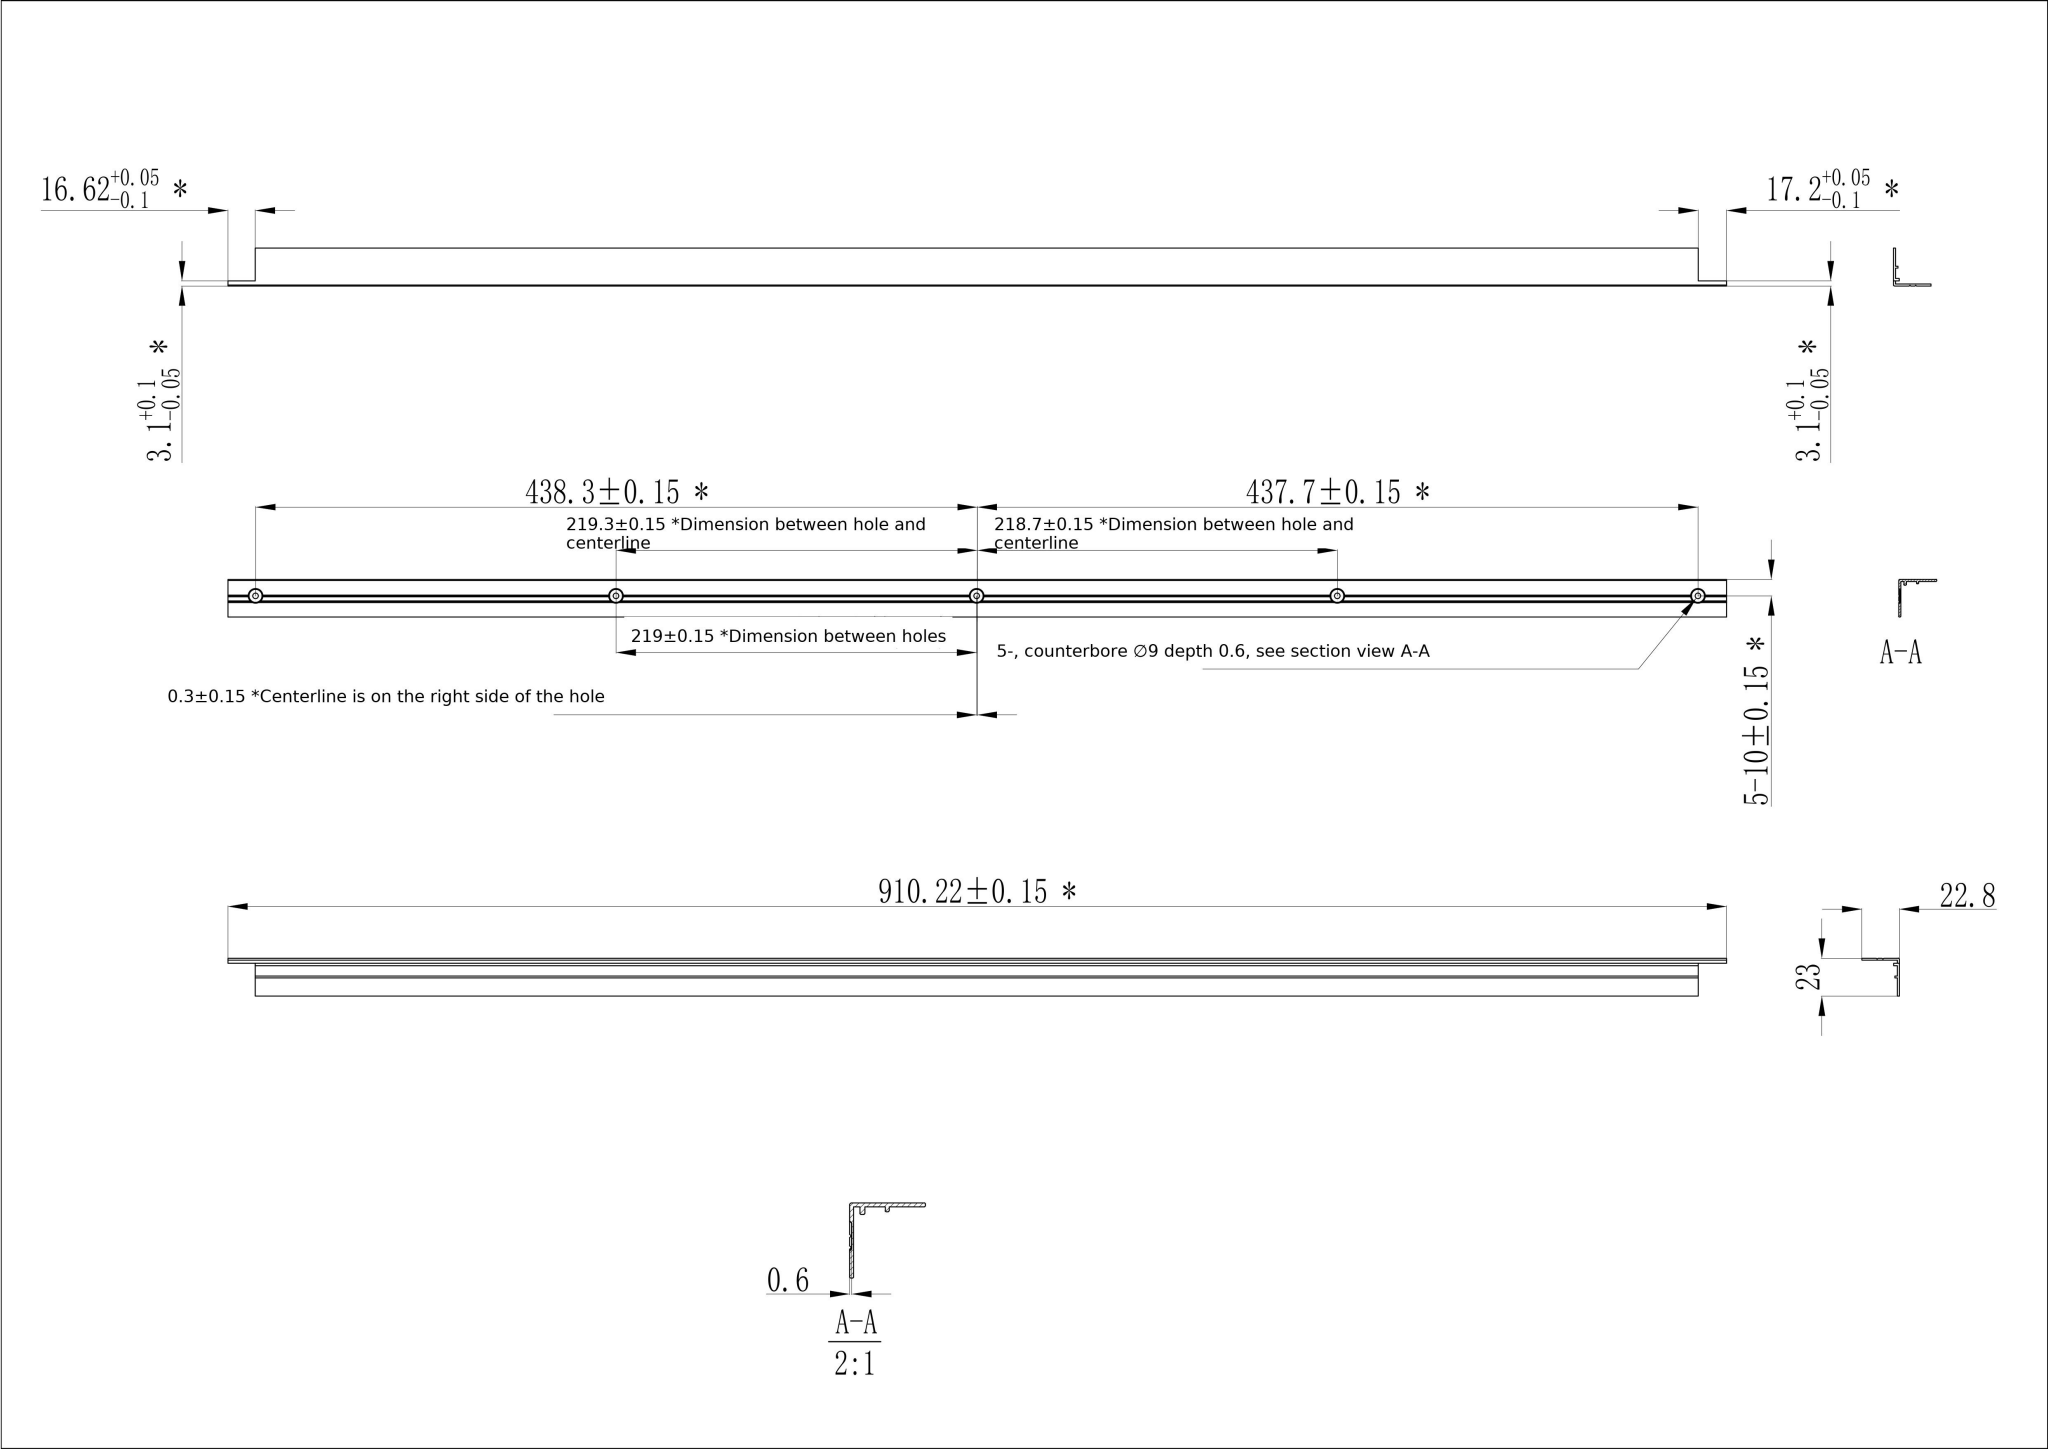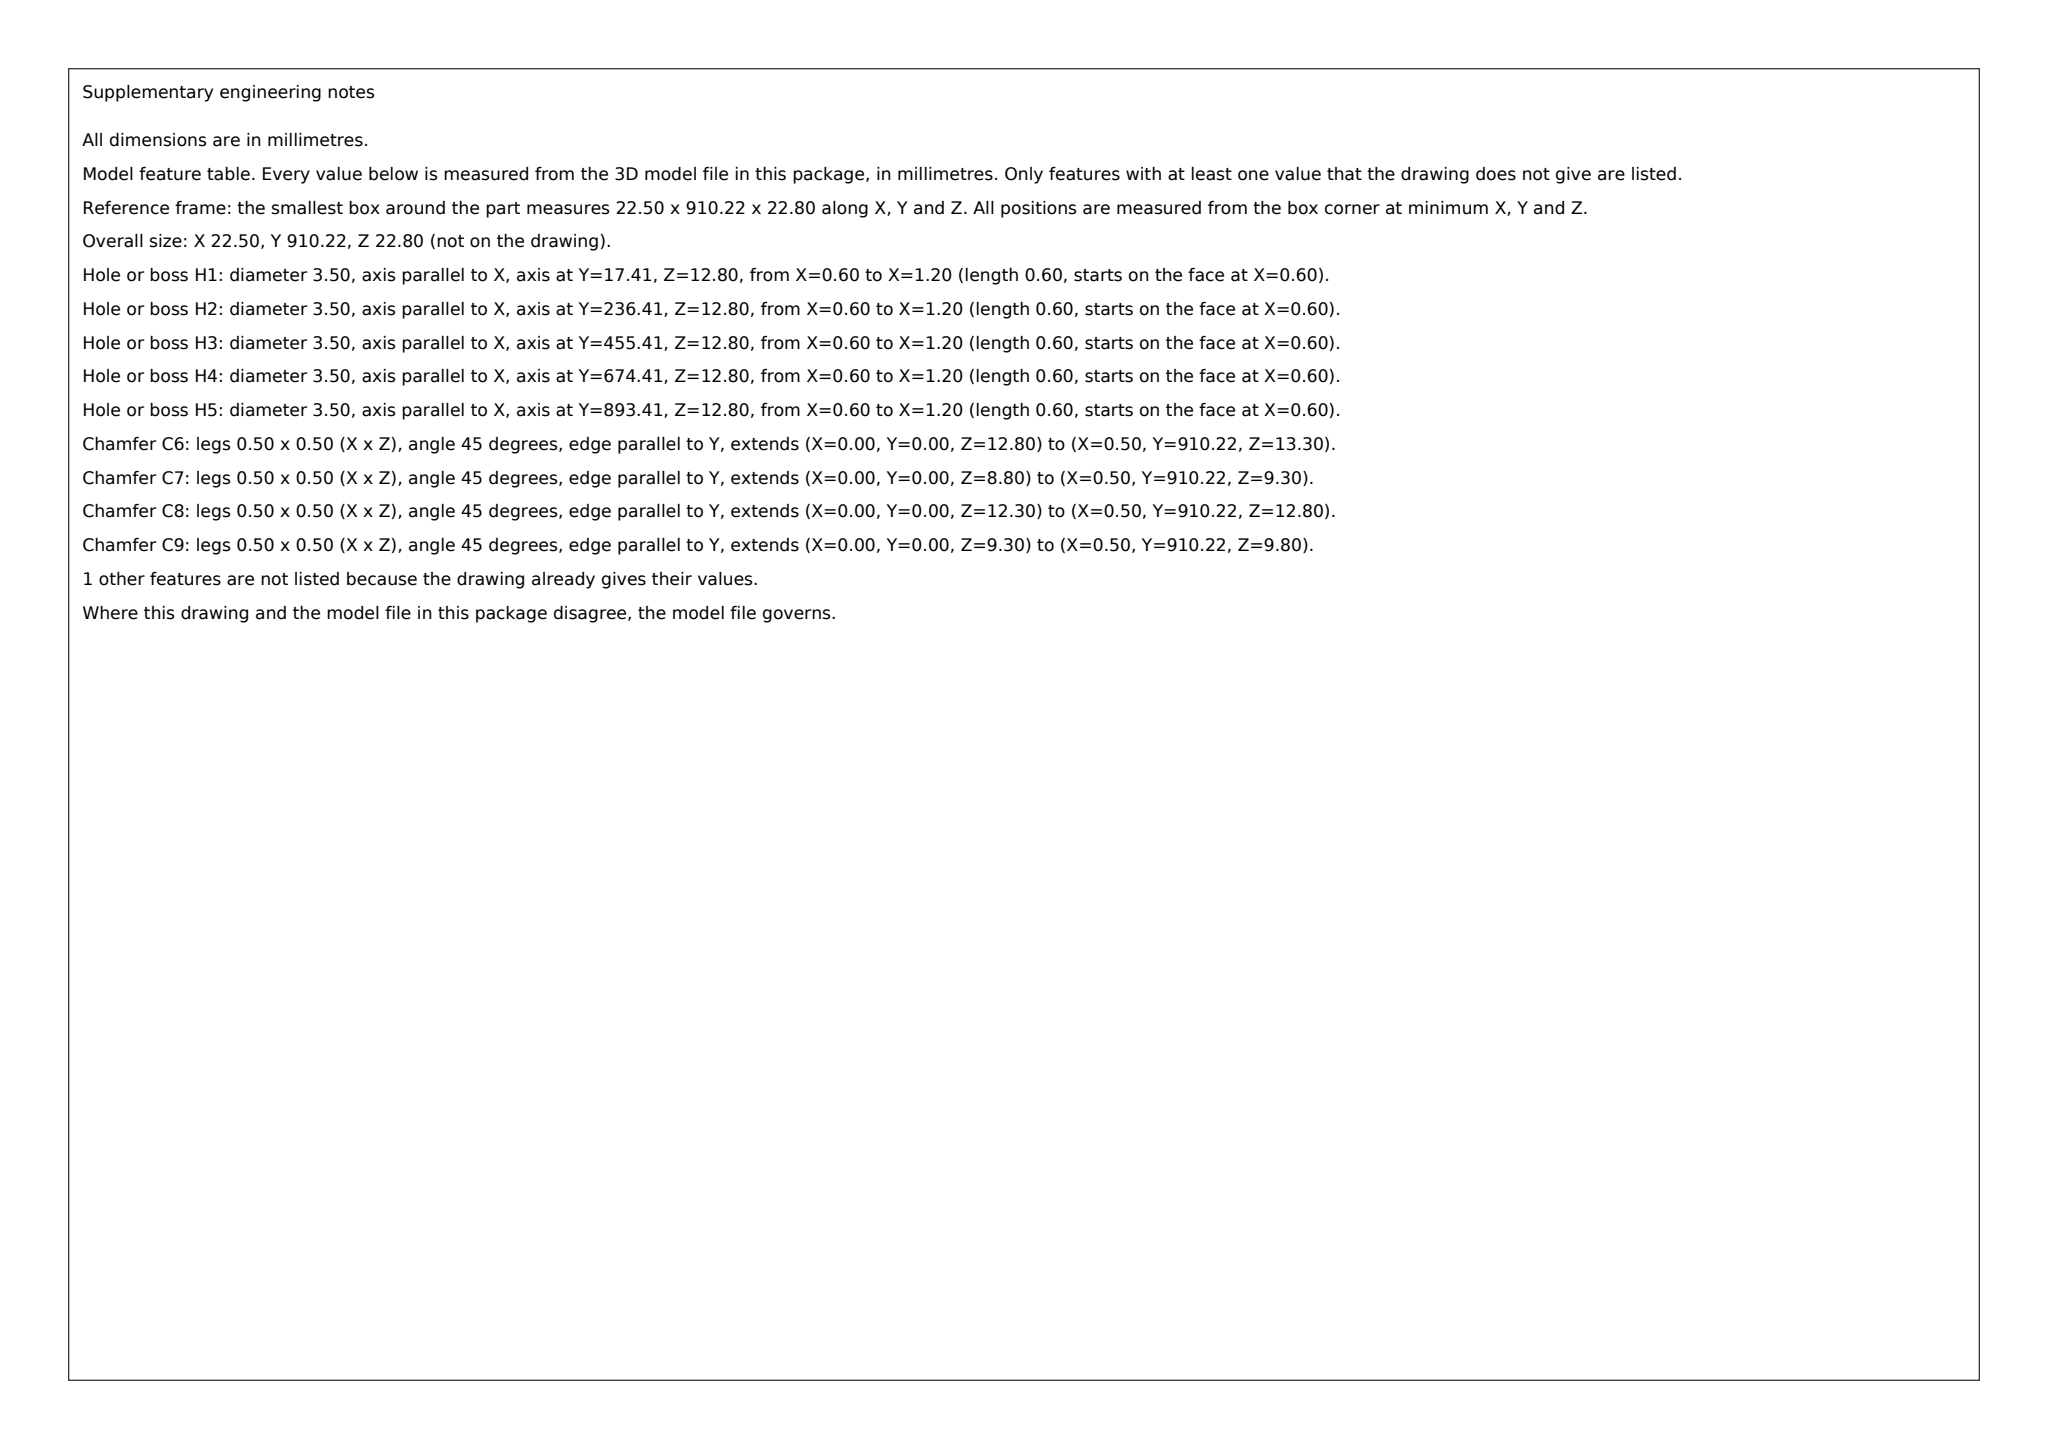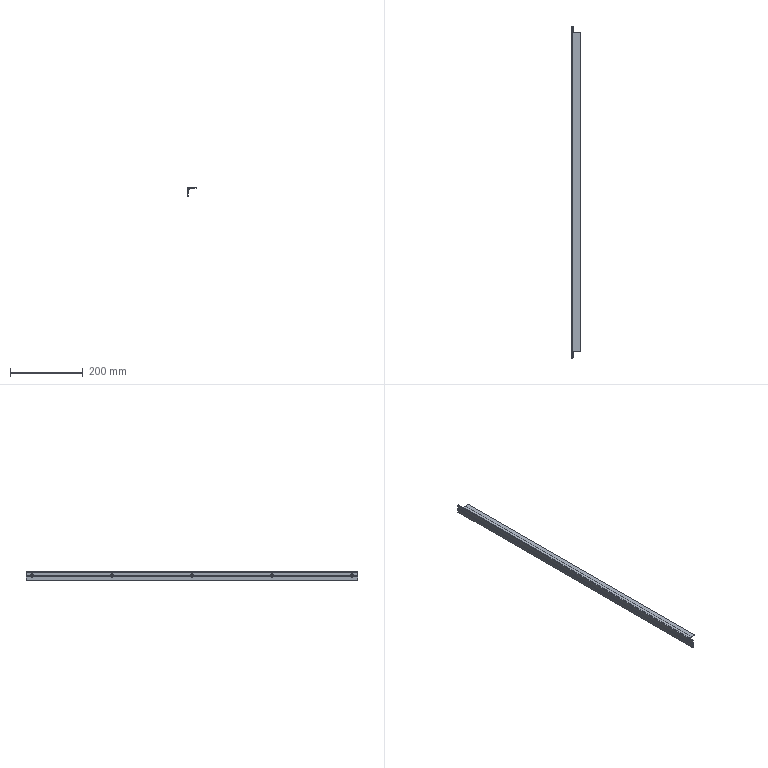Part | SolidWorks | mm | 1 solid | 77 faces | box 22.5 x 910.22 x 22.8 mm | volume 51279 mm3 | plane 56 | cylinder 11 | cone 10 | commonest cylinder face diameters 3.5 x10 1.2 x1